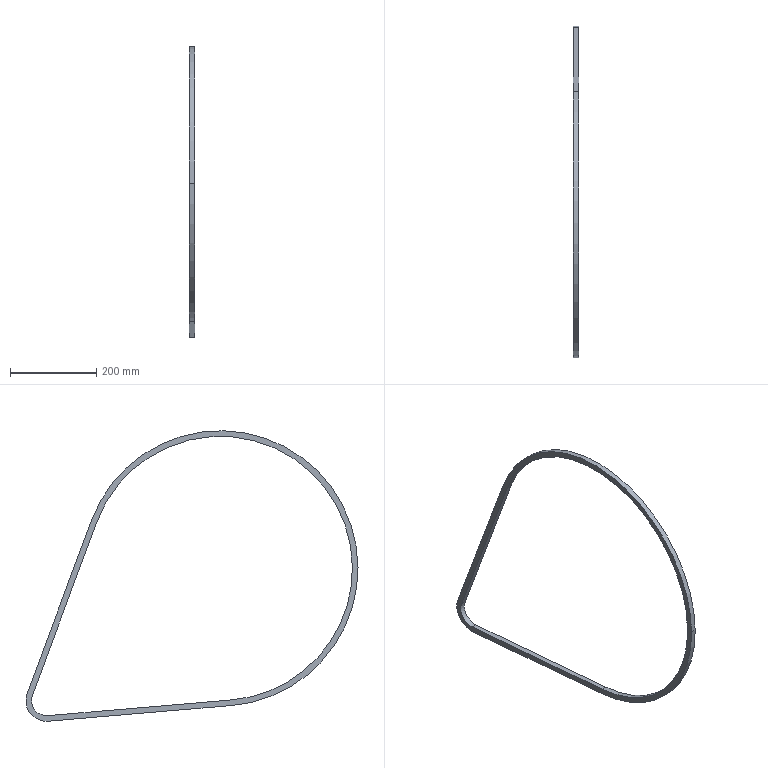Component | SolidWorks | Belt-3 | 1 solid | 12 faces | box 12 x 772.27 x 675.6 mm | volume 355790 mm3 | cylinder 6 | plane 6 | commonest cylinder face diameters 614 x2 640 x2 96 x1 70 x1
build123d program:
from build123d import *

# Parameters (mm, degrees)
BOSS_EXTRUDE1_DEPTH = 12


with BuildPart() as part:
    # Sketch1 → Boss-Extrude1 (new body)
    with BuildSketch(Plane(origin=(0, 0, 15.778), x_dir=(-1, 0, 0), z_dir=(0, 0, -1))):
        with BuildLine():
            Line((-45.803, 15.2), (106.962, 416.112))
            ThreePointArc((106.962, 416.112), (662.334, 493.71), (430.499, -16.89))
            Line((430.499, -16.89), (2.728, -49.75))
            ThreePointArc((2.728, -49.75), (-39.4, -30.622), (-45.803, 15.2))
        make_face()
        with BuildLine():
            Line((-33.655, 10.571), (119.11, 411.483))
            ThreePointArc((119.11, 411.483), (651.92, 485.929), (429.503, -3.928))
            Line((429.503, -3.928), (1.732, -36.788))
            ThreePointArc((1.732, -36.788), (-28.986, -22.841), (-33.655, 10.571))
        make_face(mode=Mode.SUBTRACT)
    extrude(amount=-BOSS_EXTRUDE1_DEPTH)


solid = part.part

# Placed as in the assembly
solid = solid.moved(Location((-852.797, 1739.103, 708.896), (89.5, 90, 0)))
STEP:
#1=COLOUR_RGB('',0.7922,0.8196,0.9333);
#2=FILL_AREA_STYLE_COLOUR('',#1);
#3=FILL_AREA_STYLE('',(#2));
#4=SURFACE_STYLE_FILL_AREA(#3);
#5=SURFACE_SIDE_STYLE('',(#4));
#6=SURFACE_STYLE_USAGE(.BOTH.,#5);
#7=PRESENTATION_STYLE_ASSIGNMENT((#6));
#8=CARTESIAN_POINT('',(-32.481,40.503,40.05));
#9=VERTEX_POINT('',#8);
#10=CARTESIAN_POINT('',(-32.481,63.921,44.15));
#11=VERTEX_POINT('',#10);
#12=CARTESIAN_POINT('',(-32.481,52.589,39.945));
#13=DIRECTION('',(-1.,0.,0.));
#14=DIRECTION('',(0.,1.,-0.008727));
#15=AXIS2_PLACEMENT_3D('',#12,#13,#14);
#16=CIRCLE('',#15,12.087);
#17=EDGE_CURVE('',#9,#11,#16,.T.);
#18=ORIENTED_EDGE('',*,*,#17,.F.);
#19=CARTESIAN_POINT('',(-32.953,40.503,40.05));
#20=VERTEX_POINT('',#19);
#21=CARTESIAN_POINT('',(-32.481,40.503,40.05));
#22=DIRECTION('',(-1.,0.,0.));
#23=VECTOR('',#22,39.37);
#24=LINE('',#21,#23);
#25=EDGE_CURVE('',#9,#20,#24,.T.);
#26=ORIENTED_EDGE('',*,*,#25,.T.);
#27=CARTESIAN_POINT('',(-32.953,63.921,44.15));
#28=VERTEX_POINT('',#27);
#29=CARTESIAN_POINT('',(-32.953,52.589,39.945));
#30=DIRECTION('',(-1.,0.,0.));
#31=DIRECTION('',(0.,1.,-0.008727));
#32=AXIS2_PLACEMENT_3D('',#29,#30,#31);
#33=CIRCLE('',#32,12.087);
#34=EDGE_CURVE('',#20,#28,#33,.T.);
#35=ORIENTED_EDGE('',*,*,#34,.T.);
#36=CARTESIAN_POINT('',(-32.481,63.921,44.15));
#37=DIRECTION('',(-1.,0.,0.));
#38=VECTOR('',#37,39.37);
#39=LINE('',#36,#38);
#40=EDGE_CURVE('',#11,#28,#39,.T.);
#41=ORIENTED_EDGE('',*,*,#40,.F.);
#42=EDGE_LOOP('',(#18,#26,#35,#41));
#43=FACE_OUTER_BOUND('',#42,.T.);
#44=CARTESIAN_POINT('',(-32.481,52.589,39.945));
#45=DIRECTION('',(-1.,0.,0.));
#46=DIRECTION('',(0.,-1.,0.008727));
#47=AXIS2_PLACEMENT_3D('',#44,#45,#46);
#48=CYLINDRICAL_SURFACE('',#47,12.087);
#49=ADVANCED_FACE('',(#43),#48,.F.);
#50=CARTESIAN_POINT('',(-32.481,51.515,27.392));
#51=VERTEX_POINT('',#50);
#52=CARTESIAN_POINT('',(-32.481,39.991,40.055));
#53=VERTEX_POINT('',#52);
#54=CARTESIAN_POINT('',(-32.481,52.589,39.945));
#55=DIRECTION('',(-1.,0.,0.));
#56=DIRECTION('',(0.,1.,-0.008727));
#57=AXIS2_PLACEMENT_3D('',#54,#55,#56);
#58=CIRCLE('',#57,12.598);
#59=EDGE_CURVE('',#51,#53,#58,.T.);
#60=ORIENTED_EDGE('',*,*,#59,.T.);
#61=CARTESIAN_POINT('',(-32.953,39.991,40.055));
#62=VERTEX_POINT('',#61);
#63=CARTESIAN_POINT('',(-32.481,39.991,40.055));
#64=DIRECTION('',(-1.,0.,0.));
#65=VECTOR('',#64,39.37);
#66=LINE('',#63,#65);
#67=EDGE_CURVE('',#53,#62,#66,.T.);
#68=ORIENTED_EDGE('',*,*,#67,.T.);
#69=CARTESIAN_POINT('',(-32.953,51.515,27.392));
#70=VERTEX_POINT('',#69);
#71=CARTESIAN_POINT('',(-32.953,52.589,39.945));
#72=DIRECTION('',(-1.,0.,0.));
#73=DIRECTION('',(0.,1.,-0.008727));
#74=AXIS2_PLACEMENT_3D('',#71,#72,#73);
#75=CIRCLE('',#74,12.598);
#76=EDGE_CURVE('',#70,#62,#75,.T.);
#77=ORIENTED_EDGE('',*,*,#76,.F.);
#78=CARTESIAN_POINT('',(-32.481,51.515,27.392));
#79=DIRECTION('',(-1.,0.,0.));
#80=VECTOR('',#79,39.37);
#81=LINE('',#78,#80);
#82=EDGE_CURVE('',#51,#70,#81,.T.);
#83=ORIENTED_EDGE('',*,*,#82,.F.);
#84=EDGE_LOOP('',(#60,#68,#77,#83));
#85=FACE_OUTER_BOUND('',#84,.T.);
#86=CARTESIAN_POINT('',(-32.481,52.589,39.945));
#87=DIRECTION('',(-1.,0.,0.));
#88=DIRECTION('',(0.,-1.,0.008727));
#89=AXIS2_PLACEMENT_3D('',#86,#87,#88);
#90=CYLINDRICAL_SURFACE('',#89,12.598);
#91=ADVANCED_FACE('',(#85),#90,.T.);
#92=CARTESIAN_POINT('',(-32.953,70.277,28.492));
#93=VERTEX_POINT('',#92);
#94=CARTESIAN_POINT('',(-32.953,68.344,25.952));
#95=VERTEX_POINT('',#94);
#96=CARTESIAN_POINT('',(-32.953,68.505,27.834));
#97=DIRECTION('',(-1.,0.,0.));
#98=DIRECTION('',(0.,1.,-0.008727));
#99=AXIS2_PLACEMENT_3D('',#96,#97,#98);
#100=CIRCLE('',#99,1.89);
#101=EDGE_CURVE('',#93,#95,#100,.T.);
#102=ORIENTED_EDGE('',*,*,#101,.F.);
#103=CARTESIAN_POINT('',(-32.481,70.277,28.492));
#104=VERTEX_POINT('',#103);
#105=CARTESIAN_POINT('',(-32.481,70.277,28.492));
#106=DIRECTION('',(-1.,0.,0.));
#107=VECTOR('',#106,39.37);
#108=LINE('',#105,#107);
#109=EDGE_CURVE('',#104,#93,#108,.T.);
#110=ORIENTED_EDGE('',*,*,#109,.F.);
#111=CARTESIAN_POINT('',(-32.481,68.344,25.952));
#112=VERTEX_POINT('',#111);
#113=CARTESIAN_POINT('',(-32.481,68.505,27.834));
#114=DIRECTION('',(-1.,0.,0.));
#115=DIRECTION('',(0.,1.,-0.008727));
#116=AXIS2_PLACEMENT_3D('',#113,#114,#115);
#117=CIRCLE('',#116,1.89);
#118=EDGE_CURVE('',#104,#112,#117,.T.);
#119=ORIENTED_EDGE('',*,*,#118,.T.);
#120=CARTESIAN_POINT('',(-32.481,68.344,25.952));
#121=DIRECTION('',(-1.,0.,0.));
#122=VECTOR('',#121,39.37);
#123=LINE('',#120,#122);
#124=EDGE_CURVE('',#112,#95,#123,.T.);
#125=ORIENTED_EDGE('',*,*,#124,.T.);
#126=EDGE_LOOP('',(#102,#110,#119,#125));
#127=FACE_OUTER_BOUND('',#126,.T.);
#128=CARTESIAN_POINT('',(-32.481,68.505,27.834));
#129=DIRECTION('',(-1.,0.,0.));
#130=DIRECTION('',(0.,-1.,0.008727));
#131=AXIS2_PLACEMENT_3D('',#128,#129,#130);
#132=CYLINDRICAL_SURFACE('',#131,1.89);
#133=ADVANCED_FACE('',(#127),#132,.T.);
#134=CARTESIAN_POINT('',(-32.953,64.401,44.328));
#135=VERTEX_POINT('',#134);
#136=CARTESIAN_POINT('',(-32.953,70.277,28.492));
#137=DIRECTION('',(0.,0.3479,-0.9375));
#138=VECTOR('',#137,39.37);
#139=LINE('',#136,#138);
#140=EDGE_CURVE('',#135,#93,#139,.T.);
#141=ORIENTED_EDGE('',*,*,#140,.F.);
#142=CARTESIAN_POINT('',(-32.481,64.401,44.328));
#143=VERTEX_POINT('',#142);
#144=CARTESIAN_POINT('',(-32.481,64.401,44.328));
#145=DIRECTION('',(-1.,0.,0.));
#146=VECTOR('',#145,39.37);
#147=LINE('',#144,#146);
#148=EDGE_CURVE('',#143,#135,#147,.T.);
#149=ORIENTED_EDGE('',*,*,#148,.F.);
#150=CARTESIAN_POINT('',(-32.481,70.277,28.492));
#151=DIRECTION('',(0.,0.3479,-0.9375));
#152=VECTOR('',#151,39.37);
#153=LINE('',#150,#152);
#154=EDGE_CURVE('',#143,#104,#153,.T.);
#155=ORIENTED_EDGE('',*,*,#154,.T.);
#156=ORIENTED_EDGE('',*,*,#109,.T.);
#157=EDGE_LOOP('',(#141,#149,#155,#156));
#158=FACE_OUTER_BOUND('',#157,.T.);
#159=CARTESIAN_POINT('',(-32.481,70.277,28.492));
#160=DIRECTION('',(0.,0.9375,0.3479));
#161=DIRECTION('',(0.,-0.3479,0.9375));
#162=AXIS2_PLACEMENT_3D('',#159,#160,#161);
#163=PLANE('',#162);
#164=ADVANCED_FACE('',(#158),#163,.T.);
#165=ORIENTED_EDGE('',*,*,#67,.F.);
#166=CARTESIAN_POINT('',(-32.481,52.589,39.945));
#167=DIRECTION('',(-1.,0.,0.));
#168=DIRECTION('',(0.,1.,-0.008727));
#169=AXIS2_PLACEMENT_3D('',#166,#167,#168);
#170=CIRCLE('',#169,12.598);
#171=EDGE_CURVE('',#53,#143,#170,.T.);
#172=ORIENTED_EDGE('',*,*,#171,.T.);
#173=ORIENTED_EDGE('',*,*,#148,.T.);
#174=CARTESIAN_POINT('',(-32.953,52.589,39.945));
#175=DIRECTION('',(-1.,0.,0.));
#176=DIRECTION('',(0.,1.,-0.008727));
#177=AXIS2_PLACEMENT_3D('',#174,#175,#176);
#178=CIRCLE('',#177,12.598);
#179=EDGE_CURVE('',#62,#135,#178,.T.);
#180=ORIENTED_EDGE('',*,*,#179,.F.);
#181=EDGE_LOOP('',(#165,#172,#173,#180));
#182=FACE_OUTER_BOUND('',#181,.T.);
#183=CARTESIAN_POINT('',(-32.481,52.589,39.945));
#184=DIRECTION('',(-1.,0.,0.));
#185=DIRECTION('',(0.,-1.,0.008727));
#186=AXIS2_PLACEMENT_3D('',#183,#184,#185);
#187=CYLINDRICAL_SURFACE('',#186,12.598);
#188=ADVANCED_FACE('',(#182),#187,.T.);
#189=CARTESIAN_POINT('',(-32.953,51.515,27.392));
#190=DIRECTION('',(0.,-0.9964,0.08529));
#191=VECTOR('',#190,39.37);
#192=LINE('',#189,#191);
#193=EDGE_CURVE('',#95,#70,#192,.T.);
#194=ORIENTED_EDGE('',*,*,#193,.F.);
#195=ORIENTED_EDGE('',*,*,#124,.F.);
#196=CARTESIAN_POINT('',(-32.481,51.515,27.392));
#197=DIRECTION('',(0.,-0.9964,0.08529));
#198=VECTOR('',#197,39.37);
#199=LINE('',#196,#198);
#200=EDGE_CURVE('',#112,#51,#199,.T.);
#201=ORIENTED_EDGE('',*,*,#200,.T.);
#202=ORIENTED_EDGE('',*,*,#82,.T.);
#203=EDGE_LOOP('',(#194,#195,#201,#202));
#204=FACE_OUTER_BOUND('',#203,.T.);
#205=CARTESIAN_POINT('',(-32.481,51.515,27.392));
#206=DIRECTION('',(0.,-0.08529,-0.9964));
#207=DIRECTION('',(0.,0.9964,-0.08529));
#208=AXIS2_PLACEMENT_3D('',#205,#206,#207);
#209=PLANE('',#208);
#210=ADVANCED_FACE('',(#204),#209,.T.);
#211=CARTESIAN_POINT('',(-32.481,69.797,28.314));
#212=VERTEX_POINT('',#211);
#213=CARTESIAN_POINT('',(-32.481,68.388,26.462));
#214=VERTEX_POINT('',#213);
#215=CARTESIAN_POINT('',(-32.481,68.505,27.834));
#216=DIRECTION('',(-1.,0.,0.));
#217=DIRECTION('',(0.,1.,-0.008727));
#218=AXIS2_PLACEMENT_3D('',#215,#216,#217);
#219=CIRCLE('',#218,1.378);
#220=EDGE_CURVE('',#212,#214,#219,.T.);
#221=ORIENTED_EDGE('',*,*,#220,.T.);
#222=CARTESIAN_POINT('',(-32.481,51.558,27.902));
#223=VERTEX_POINT('',#222);
#224=CARTESIAN_POINT('',(-32.481,51.558,27.902));
#225=DIRECTION('',(0.,-0.9964,0.08529));
#226=VECTOR('',#225,39.37);
#227=LINE('',#224,#226);
#228=EDGE_CURVE('',#214,#223,#227,.T.);
#229=ORIENTED_EDGE('',*,*,#228,.T.);
#230=CARTESIAN_POINT('',(-32.481,52.589,39.945));
#231=DIRECTION('',(-1.,0.,0.));
#232=DIRECTION('',(0.,1.,-0.008727));
#233=AXIS2_PLACEMENT_3D('',#230,#231,#232);
#234=CIRCLE('',#233,12.087);
#235=EDGE_CURVE('',#223,#9,#234,.T.);
#236=ORIENTED_EDGE('',*,*,#235,.T.);
#237=ORIENTED_EDGE('',*,*,#17,.T.);
#238=CARTESIAN_POINT('',(-32.481,69.797,28.314));
#239=DIRECTION('',(0.,0.3479,-0.9375));
#240=VECTOR('',#239,39.37);
#241=LINE('',#238,#240);
#242=EDGE_CURVE('',#11,#212,#241,.T.);
#243=ORIENTED_EDGE('',*,*,#242,.T.);
#244=EDGE_LOOP('',(#221,#229,#236,#237,#243));
#245=FACE_BOUND('',#244,.T.);
#246=ORIENTED_EDGE('',*,*,#118,.F.);
#247=ORIENTED_EDGE('',*,*,#154,.F.);
#248=ORIENTED_EDGE('',*,*,#171,.F.);
#249=ORIENTED_EDGE('',*,*,#59,.F.);
#250=ORIENTED_EDGE('',*,*,#200,.F.);
#251=EDGE_LOOP('',(#246,#247,#248,#249,#250));
#252=FACE_OUTER_BOUND('',#251,.T.);
#253=CARTESIAN_POINT('',(-32.481,68.505,27.834));
#254=DIRECTION('',(1.,0.,0.));
#255=DIRECTION('',(0.,1.,-0.008727));
#256=AXIS2_PLACEMENT_3D('',#253,#254,#255);
#257=PLANE('',#256);
#258=ADVANCED_FACE('',(#245,#252),#257,.T.);
#259=CARTESIAN_POINT('',(-32.953,68.388,26.462));
#260=VERTEX_POINT('',#259);
#261=CARTESIAN_POINT('',(-32.953,51.558,27.902));
#262=VERTEX_POINT('',#261);
#263=CARTESIAN_POINT('',(-32.953,51.558,27.902));
#264=DIRECTION('',(0.,-0.9964,0.08529));
#265=VECTOR('',#264,39.37);
#266=LINE('',#263,#265);
#267=EDGE_CURVE('',#260,#262,#266,.T.);
#268=ORIENTED_EDGE('',*,*,#267,.F.);
#269=CARTESIAN_POINT('',(-32.953,69.797,28.314));
#270=VERTEX_POINT('',#269);
#271=CARTESIAN_POINT('',(-32.953,68.505,27.834));
#272=DIRECTION('',(-1.,0.,0.));
#273=DIRECTION('',(0.,1.,-0.008727));
#274=AXIS2_PLACEMENT_3D('',#271,#272,#273);
#275=CIRCLE('',#274,1.378);
#276=EDGE_CURVE('',#270,#260,#275,.T.);
#277=ORIENTED_EDGE('',*,*,#276,.F.);
#278=CARTESIAN_POINT('',(-32.953,69.797,28.314));
#279=DIRECTION('',(0.,0.3479,-0.9375));
#280=VECTOR('',#279,39.37);
#281=LINE('',#278,#280);
#282=EDGE_CURVE('',#28,#270,#281,.T.);
#283=ORIENTED_EDGE('',*,*,#282,.F.);
#284=ORIENTED_EDGE('',*,*,#34,.F.);
#285=CARTESIAN_POINT('',(-32.953,52.589,39.945));
#286=DIRECTION('',(-1.,0.,0.));
#287=DIRECTION('',(0.,1.,-0.008727));
#288=AXIS2_PLACEMENT_3D('',#285,#286,#287);
#289=CIRCLE('',#288,12.087);
#290=EDGE_CURVE('',#262,#20,#289,.T.);
#291=ORIENTED_EDGE('',*,*,#290,.F.);
#292=EDGE_LOOP('',(#268,#277,#283,#284,#291));
#293=FACE_BOUND('',#292,.T.);
#294=ORIENTED_EDGE('',*,*,#101,.T.);
#295=ORIENTED_EDGE('',*,*,#193,.T.);
#296=ORIENTED_EDGE('',*,*,#76,.T.);
#297=ORIENTED_EDGE('',*,*,#179,.T.);
#298=ORIENTED_EDGE('',*,*,#140,.T.);
#299=EDGE_LOOP('',(#294,#295,#296,#297,#298));
#300=FACE_OUTER_BOUND('',#299,.T.);
#301=CARTESIAN_POINT('',(-32.953,68.505,27.834));
#302=DIRECTION('',(1.,0.,0.));
#303=DIRECTION('',(0.,1.,-0.008727));
#304=AXIS2_PLACEMENT_3D('',#301,#302,#303);
#305=PLANE('',#304);
#306=ADVANCED_FACE('',(#293,#300),#305,.F.);
#307=ORIENTED_EDGE('',*,*,#276,.T.);
#308=CARTESIAN_POINT('',(-32.481,68.388,26.462));
#309=DIRECTION('',(-1.,0.,0.));
#310=VECTOR('',#309,39.37);
#311=LINE('',#308,#310);
#312=EDGE_CURVE('',#214,#260,#311,.T.);
#313=ORIENTED_EDGE('',*,*,#312,.F.);
#314=ORIENTED_EDGE('',*,*,#220,.F.);
#315=CARTESIAN_POINT('',(-32.481,69.797,28.314));
#316=DIRECTION('',(-1.,0.,0.));
#317=VECTOR('',#316,39.37);
#318=LINE('',#315,#317);
#319=EDGE_CURVE('',#212,#270,#318,.T.);
#320=ORIENTED_EDGE('',*,*,#319,.T.);
#321=EDGE_LOOP('',(#307,#313,#314,#320));
#322=FACE_OUTER_BOUND('',#321,.T.);
#323=CARTESIAN_POINT('',(-32.481,68.505,27.834));
#324=DIRECTION('',(-1.,0.,0.));
#325=DIRECTION('',(0.,-1.,0.008727));
#326=AXIS2_PLACEMENT_3D('',#323,#324,#325);
#327=CYLINDRICAL_SURFACE('',#326,1.378);
#328=ADVANCED_FACE('',(#322),#327,.F.);
#329=ORIENTED_EDGE('',*,*,#282,.T.);
#330=ORIENTED_EDGE('',*,*,#319,.F.);
#331=ORIENTED_EDGE('',*,*,#242,.F.);
#332=ORIENTED_EDGE('',*,*,#40,.T.);
#333=EDGE_LOOP('',(#329,#330,#331,#332));
#334=FACE_OUTER_BOUND('',#333,.T.);
#335=CARTESIAN_POINT('',(-32.481,69.797,28.314));
#336=DIRECTION('',(0.,0.9375,0.3479));
#337=DIRECTION('',(0.,-0.3479,0.9375));
#338=AXIS2_PLACEMENT_3D('',#335,#336,#337);
#339=PLANE('',#338);
#340=ADVANCED_FACE('',(#334),#339,.F.);
#341=ORIENTED_EDGE('',*,*,#25,.F.);
#342=ORIENTED_EDGE('',*,*,#235,.F.);
#343=CARTESIAN_POINT('',(-32.481,51.558,27.902));
#344=DIRECTION('',(-1.,0.,0.));
#345=VECTOR('',#344,39.37);
#346=LINE('',#343,#345);
#347=EDGE_CURVE('',#223,#262,#346,.T.);
#348=ORIENTED_EDGE('',*,*,#347,.T.);
#349=ORIENTED_EDGE('',*,*,#290,.T.);
#350=EDGE_LOOP('',(#341,#342,#348,#349));
#351=FACE_OUTER_BOUND('',#350,.T.);
#352=CARTESIAN_POINT('',(-32.481,52.589,39.945));
#353=DIRECTION('',(-1.,0.,0.));
#354=DIRECTION('',(0.,-1.,0.008727));
#355=AXIS2_PLACEMENT_3D('',#352,#353,#354);
#356=CYLINDRICAL_SURFACE('',#355,12.087);
#357=ADVANCED_FACE('',(#351),#356,.F.);
#358=ORIENTED_EDGE('',*,*,#267,.T.);
#359=ORIENTED_EDGE('',*,*,#347,.F.);
#360=ORIENTED_EDGE('',*,*,#228,.F.);
#361=ORIENTED_EDGE('',*,*,#312,.T.);
#362=EDGE_LOOP('',(#358,#359,#360,#361));
#363=FACE_OUTER_BOUND('',#362,.T.);
#364=CARTESIAN_POINT('',(-32.481,51.558,27.902));
#365=DIRECTION('',(0.,-0.08529,-0.9964));
#366=DIRECTION('',(0.,0.9964,-0.08529));
#367=AXIS2_PLACEMENT_3D('',#364,#365,#366);
#368=PLANE('',#367);
#369=ADVANCED_FACE('',(#363),#368,.F.);
#370=CLOSED_SHELL('',(#49,#91,#133,#164,#188,#210,#258,#306,#328,#340,#357,#369));
#371=MANIFOLD_SOLID_BREP('',#370);
#372=STYLED_ITEM('',(#7),#371);
#373=PRESENTATION_LAYER_ASSIGNMENT('','',(#372));
#374=CARTESIAN_POINT('',(0.,0.,0.));
#375=DIRECTION('',(0.,0.,1.));
#376=DIRECTION('',(1.,0.,0.));
#377=AXIS2_PLACEMENT_3D('',#374,#375,#376);
#378=(LENGTH_UNIT()NAMED_UNIT(*)SI_UNIT($,.METRE.));
#379=LENGTH_MEASURE_WITH_UNIT(LENGTH_MEASURE(0.0254),#378);
#380=DIMENSIONAL_EXPONENTS(1.,0.,0.,0.,0.,0.,0.);
#381=(CONVERSION_BASED_UNIT('',#379)LENGTH_UNIT()NAMED_UNIT(#380));
#382=UNCERTAINTY_MEASURE_WITH_UNIT(LENGTH_MEASURE(0.00001),#381,'','');
#383=(NAMED_UNIT(*)PLANE_ANGLE_UNIT()SI_UNIT($,.RADIAN.));
#384=(NAMED_UNIT(*)SI_UNIT($,.STERADIAN.)SOLID_ANGLE_UNIT());
#385=(GEOMETRIC_REPRESENTATION_CONTEXT(3)GLOBAL_UNCERTAINTY_ASSIGNED_CONTEXT((#382))GLOBAL_UNIT_ASSIGNED_CONTEXT((#381,#383,#384))REPRESENTATION_CONTEXT('',''));
#386=ADVANCED_BREP_SHAPE_REPRESENTATION('',(#371,#377),#385);
#387=(LENGTH_UNIT()NAMED_UNIT(*)SI_UNIT($,.METRE.));
#388=LENGTH_MEASURE_WITH_UNIT(LENGTH_MEASURE(0.0254),#387);
#389=DIMENSIONAL_EXPONENTS(1.,0.,0.,0.,0.,0.,0.);
#390=(CONVERSION_BASED_UNIT('',#388)LENGTH_UNIT()NAMED_UNIT(#389));
#391=UNCERTAINTY_MEASURE_WITH_UNIT(LENGTH_MEASURE(0.00001),#390,'','');
#392=(NAMED_UNIT(*)PLANE_ANGLE_UNIT()SI_UNIT($,.RADIAN.));
#393=(NAMED_UNIT(*)SI_UNIT($,.STERADIAN.)SOLID_ANGLE_UNIT());
#394=(GEOMETRIC_REPRESENTATION_CONTEXT(3)GLOBAL_UNCERTAINTY_ASSIGNED_CONTEXT((#391))GLOBAL_UNIT_ASSIGNED_CONTEXT((#390,#392,#393))REPRESENTATION_CONTEXT('',''));
#395=MECHANICAL_DESIGN_GEOMETRIC_PRESENTATION_REPRESENTATION('',(#372),#394);